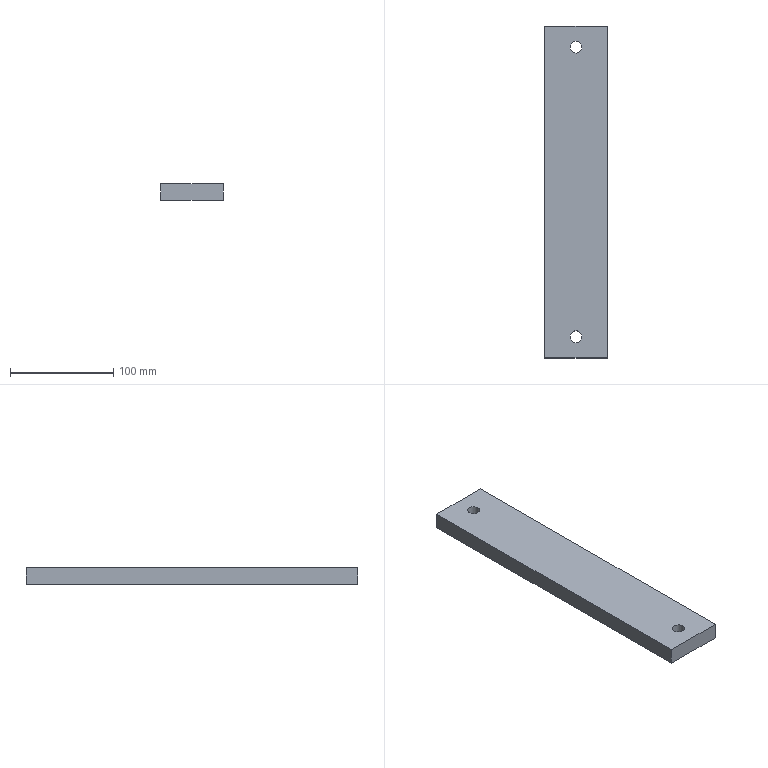Component | NX | CH3404_5-10_2 | 1 solid | 8 faces | box 60 x 321 x 16 mm | volume 304836 mm3 | plane 6 | cylinder 2 | commonest cylinder face diameters 11.5 x2
STEP:
#1=CARTESIAN_POINT('',(0.,0.,0.));
#2=DIRECTION('',(0.,0.,1.));
#3=DIRECTION('',(1.,0.,0.));
#4=AXIS2_PLACEMENT_3D('',#1,#2,#3);
#5=CARTESIAN_POINT('',(295.,-160.5,-205.));
#6=VERTEX_POINT('',#5);
#7=CARTESIAN_POINT('',(355.,-160.5,-205.));
#8=VERTEX_POINT('',#7);
#9=CARTESIAN_POINT('',(295.,-160.5,-205.));
#10=DIRECTION('',(1.,0.,0.));
#11=VECTOR('',#10,1.);
#12=LINE('',#9,#11);
#13=CARTESIAN_POINT('',(295.,-160.5,-189.));
#14=DIRECTION('',(0.,1.,0.));
#15=DIRECTION('',(0.,0.,-1.));
#16=AXIS2_PLACEMENT_3D('',#13,#14,#15);
#17=PLANE('',#16);
#18=CARTESIAN_POINT('',(16.,0.));
#19=DIRECTION('',(0.,-1.));
#20=VECTOR('',#19,1.);
#21=LINE('',#18,#20);
#22=(GEOMETRIC_REPRESENTATION_CONTEXT(2)PARAMETRIC_REPRESENTATION_CONTEXT()REPRESENTATION_CONTEXT('',''));
#23=DEFINITIONAL_REPRESENTATION('',(#21),#22);
#24=PCURVE('',#17,#23);
#25=CARTESIAN_POINT('',(325.,0.,-205.));
#26=DIRECTION('',(0.,0.,1.));
#27=DIRECTION('',(0.,1.,0.));
#28=AXIS2_PLACEMENT_3D('',#25,#26,#27);
#29=PLANE('',#28);
#30=CARTESIAN_POINT('',(-160.5,30.));
#31=DIRECTION('',(0.,-1.));
#32=VECTOR('',#31,1.);
#33=LINE('',#30,#32);
#34=(GEOMETRIC_REPRESENTATION_CONTEXT(2)PARAMETRIC_REPRESENTATION_CONTEXT()REPRESENTATION_CONTEXT('',''));
#35=DEFINITIONAL_REPRESENTATION('',(#33),#34);
#36=PCURVE('',#29,#35);
#37=SURFACE_CURVE('',#12,(#24,#36),.PCURVE_S1.);
#38=EDGE_CURVE('',#6,#8,#37,.T.);
#39=ORIENTED_EDGE('',*,*,#38,.T.);
#40=CARTESIAN_POINT('',(355.,-160.5,-189.));
#41=VERTEX_POINT('',#40);
#42=CARTESIAN_POINT('',(355.,-160.5,-189.));
#43=DIRECTION('',(0.,0.,-1.));
#44=VECTOR('',#43,1.);
#45=LINE('',#42,#44);
#46=CARTESIAN_POINT('',(0.,-60.));
#47=DIRECTION('',(1.,0.));
#48=VECTOR('',#47,1.);
#49=LINE('',#46,#48);
#50=(GEOMETRIC_REPRESENTATION_CONTEXT(2)PARAMETRIC_REPRESENTATION_CONTEXT()REPRESENTATION_CONTEXT('',''));
#51=DEFINITIONAL_REPRESENTATION('',(#49),#50);
#52=PCURVE('',#17,#51);
#53=CARTESIAN_POINT('',(355.,-160.5,-189.));
#54=DIRECTION('',(-1.,0.,0.));
#55=DIRECTION('',(0.,0.,1.));
#56=AXIS2_PLACEMENT_3D('',#53,#54,#55);
#57=PLANE('',#56);
#58=CARTESIAN_POINT('',(0.,0.));
#59=DIRECTION('',(-1.,0.));
#60=VECTOR('',#59,1.);
#61=LINE('',#58,#60);
#62=(GEOMETRIC_REPRESENTATION_CONTEXT(2)PARAMETRIC_REPRESENTATION_CONTEXT()REPRESENTATION_CONTEXT('',''));
#63=DEFINITIONAL_REPRESENTATION('',(#61),#62);
#64=PCURVE('',#57,#63);
#65=SURFACE_CURVE('',#45,(#52,#64),.PCURVE_S1.);
#66=EDGE_CURVE('',#41,#8,#65,.T.);
#67=ORIENTED_EDGE('',*,*,#66,.F.);
#68=CARTESIAN_POINT('',(295.,-160.5,-189.));
#69=VERTEX_POINT('',#68);
#70=CARTESIAN_POINT('',(295.,-160.5,-189.));
#71=DIRECTION('',(1.,0.,0.));
#72=VECTOR('',#71,1.);
#73=LINE('',#70,#72);
#74=CARTESIAN_POINT('',(0.,0.));
#75=DIRECTION('',(0.,-1.));
#76=VECTOR('',#75,1.);
#77=LINE('',#74,#76);
#78=(GEOMETRIC_REPRESENTATION_CONTEXT(2)PARAMETRIC_REPRESENTATION_CONTEXT()REPRESENTATION_CONTEXT('',''));
#79=DEFINITIONAL_REPRESENTATION('',(#77),#78);
#80=PCURVE('',#17,#79);
#81=CARTESIAN_POINT('',(325.,0.,-189.));
#82=DIRECTION('',(0.,0.,1.));
#83=DIRECTION('',(0.,1.,0.));
#84=AXIS2_PLACEMENT_3D('',#81,#82,#83);
#85=PLANE('',#84);
#86=CARTESIAN_POINT('',(-160.5,30.));
#87=DIRECTION('',(0.,-1.));
#88=VECTOR('',#87,1.);
#89=LINE('',#86,#88);
#90=(GEOMETRIC_REPRESENTATION_CONTEXT(2)PARAMETRIC_REPRESENTATION_CONTEXT()REPRESENTATION_CONTEXT('',''));
#91=DEFINITIONAL_REPRESENTATION('',(#89),#90);
#92=PCURVE('',#85,#91);
#93=SURFACE_CURVE('',#73,(#80,#92),.PCURVE_S1.);
#94=EDGE_CURVE('',#69,#41,#93,.T.);
#95=ORIENTED_EDGE('',*,*,#94,.F.);
#96=CARTESIAN_POINT('',(295.,-160.5,-189.));
#97=DIRECTION('',(0.,0.,-1.));
#98=VECTOR('',#97,1.);
#99=LINE('',#96,#98);
#100=CARTESIAN_POINT('',(0.,0.));
#101=DIRECTION('',(1.,0.));
#102=VECTOR('',#101,1.);
#103=LINE('',#100,#102);
#104=(GEOMETRIC_REPRESENTATION_CONTEXT(2)PARAMETRIC_REPRESENTATION_CONTEXT()REPRESENTATION_CONTEXT('',''));
#105=DEFINITIONAL_REPRESENTATION('',(#103),#104);
#106=PCURVE('',#17,#105);
#107=CARTESIAN_POINT('',(295.,160.5,-189.));
#108=DIRECTION('',(1.,0.,0.));
#109=DIRECTION('',(0.,0.,-1.));
#110=AXIS2_PLACEMENT_3D('',#107,#108,#109);
#111=PLANE('',#110);
#112=CARTESIAN_POINT('',(0.,-321.));
#113=DIRECTION('',(1.,0.));
#114=VECTOR('',#113,1.);
#115=LINE('',#112,#114);
#116=(GEOMETRIC_REPRESENTATION_CONTEXT(2)PARAMETRIC_REPRESENTATION_CONTEXT()REPRESENTATION_CONTEXT('',''));
#117=DEFINITIONAL_REPRESENTATION('',(#115),#116);
#118=PCURVE('',#111,#117);
#119=SURFACE_CURVE('',#99,(#106,#118),.PCURVE_S1.);
#120=EDGE_CURVE('',#69,#6,#119,.T.);
#121=ORIENTED_EDGE('',*,*,#120,.T.);
#122=EDGE_LOOP('',(#39,#67,#95,#121));
#123=FACE_BOUND('',#122,.T.);
#124=ADVANCED_FACE('',(#123),#17,.F.);
#125=CARTESIAN_POINT('',(355.,160.5,-205.));
#126=VERTEX_POINT('',#125);
#127=CARTESIAN_POINT('',(355.,-160.5,-205.));
#128=DIRECTION('',(0.,1.,0.));
#129=VECTOR('',#128,1.);
#130=LINE('',#127,#129);
#131=CARTESIAN_POINT('',(-16.,0.));
#132=DIRECTION('',(0.,1.));
#133=VECTOR('',#132,1.);
#134=LINE('',#131,#133);
#135=(GEOMETRIC_REPRESENTATION_CONTEXT(2)PARAMETRIC_REPRESENTATION_CONTEXT()REPRESENTATION_CONTEXT('',''));
#136=DEFINITIONAL_REPRESENTATION('',(#134),#135);
#137=PCURVE('',#57,#136);
#138=CARTESIAN_POINT('',(-160.5,-30.));
#139=DIRECTION('',(1.,0.));
#140=VECTOR('',#139,1.);
#141=LINE('',#138,#140);
#142=(GEOMETRIC_REPRESENTATION_CONTEXT(2)PARAMETRIC_REPRESENTATION_CONTEXT()REPRESENTATION_CONTEXT('',''));
#143=DEFINITIONAL_REPRESENTATION('',(#141),#142);
#144=PCURVE('',#29,#143);
#145=SURFACE_CURVE('',#130,(#137,#144),.PCURVE_S1.);
#146=EDGE_CURVE('',#8,#126,#145,.T.);
#147=ORIENTED_EDGE('',*,*,#146,.T.);
#148=CARTESIAN_POINT('',(355.,160.5,-189.));
#149=VERTEX_POINT('',#148);
#150=CARTESIAN_POINT('',(355.,160.5,-189.));
#151=DIRECTION('',(0.,0.,-1.));
#152=VECTOR('',#151,1.);
#153=LINE('',#150,#152);
#154=CARTESIAN_POINT('',(0.,321.));
#155=DIRECTION('',(-1.,0.));
#156=VECTOR('',#155,1.);
#157=LINE('',#154,#156);
#158=(GEOMETRIC_REPRESENTATION_CONTEXT(2)PARAMETRIC_REPRESENTATION_CONTEXT()REPRESENTATION_CONTEXT('',''));
#159=DEFINITIONAL_REPRESENTATION('',(#157),#158);
#160=PCURVE('',#57,#159);
#161=CARTESIAN_POINT('',(355.,160.5,-189.));
#162=DIRECTION('',(0.,-1.,0.));
#163=DIRECTION('',(0.,0.,1.));
#164=AXIS2_PLACEMENT_3D('',#161,#162,#163);
#165=PLANE('',#164);
#166=CARTESIAN_POINT('',(0.,0.));
#167=DIRECTION('',(-1.,0.));
#168=VECTOR('',#167,1.);
#169=LINE('',#166,#168);
#170=(GEOMETRIC_REPRESENTATION_CONTEXT(2)PARAMETRIC_REPRESENTATION_CONTEXT()REPRESENTATION_CONTEXT('',''));
#171=DEFINITIONAL_REPRESENTATION('',(#169),#170);
#172=PCURVE('',#165,#171);
#173=SURFACE_CURVE('',#153,(#160,#172),.PCURVE_S1.);
#174=EDGE_CURVE('',#149,#126,#173,.T.);
#175=ORIENTED_EDGE('',*,*,#174,.F.);
#176=CARTESIAN_POINT('',(355.,-160.5,-189.));
#177=DIRECTION('',(0.,1.,0.));
#178=VECTOR('',#177,1.);
#179=LINE('',#176,#178);
#180=CARTESIAN_POINT('',(0.,0.));
#181=DIRECTION('',(0.,1.));
#182=VECTOR('',#181,1.);
#183=LINE('',#180,#182);
#184=(GEOMETRIC_REPRESENTATION_CONTEXT(2)PARAMETRIC_REPRESENTATION_CONTEXT()REPRESENTATION_CONTEXT('',''));
#185=DEFINITIONAL_REPRESENTATION('',(#183),#184);
#186=PCURVE('',#57,#185);
#187=CARTESIAN_POINT('',(-160.5,-30.));
#188=DIRECTION('',(1.,0.));
#189=VECTOR('',#188,1.);
#190=LINE('',#187,#189);
#191=(GEOMETRIC_REPRESENTATION_CONTEXT(2)PARAMETRIC_REPRESENTATION_CONTEXT()REPRESENTATION_CONTEXT('',''));
#192=DEFINITIONAL_REPRESENTATION('',(#190),#191);
#193=PCURVE('',#85,#192);
#194=SURFACE_CURVE('',#179,(#186,#193),.PCURVE_S1.);
#195=EDGE_CURVE('',#41,#149,#194,.T.);
#196=ORIENTED_EDGE('',*,*,#195,.F.);
#197=ORIENTED_EDGE('',*,*,#66,.T.);
#198=EDGE_LOOP('',(#147,#175,#196,#197));
#199=FACE_BOUND('',#198,.T.);
#200=ADVANCED_FACE('',(#199),#57,.F.);
#201=CARTESIAN_POINT('',(295.,160.5,-205.));
#202=VERTEX_POINT('',#201);
#203=CARTESIAN_POINT('',(355.,160.5,-205.));
#204=DIRECTION('',(-1.,0.,0.));
#205=VECTOR('',#204,1.);
#206=LINE('',#203,#205);
#207=CARTESIAN_POINT('',(-16.,0.));
#208=DIRECTION('',(0.,1.));
#209=VECTOR('',#208,1.);
#210=LINE('',#207,#209);
#211=(GEOMETRIC_REPRESENTATION_CONTEXT(2)PARAMETRIC_REPRESENTATION_CONTEXT()REPRESENTATION_CONTEXT('',''));
#212=DEFINITIONAL_REPRESENTATION('',(#210),#211);
#213=PCURVE('',#165,#212);
#214=CARTESIAN_POINT('',(160.5,-30.));
#215=DIRECTION('',(0.,1.));
#216=VECTOR('',#215,1.);
#217=LINE('',#214,#216);
#218=(GEOMETRIC_REPRESENTATION_CONTEXT(2)PARAMETRIC_REPRESENTATION_CONTEXT()REPRESENTATION_CONTEXT('',''));
#219=DEFINITIONAL_REPRESENTATION('',(#217),#218);
#220=PCURVE('',#29,#219);
#221=SURFACE_CURVE('',#206,(#213,#220),.PCURVE_S1.);
#222=EDGE_CURVE('',#126,#202,#221,.T.);
#223=ORIENTED_EDGE('',*,*,#222,.T.);
#224=CARTESIAN_POINT('',(295.,160.5,-189.));
#225=VERTEX_POINT('',#224);
#226=CARTESIAN_POINT('',(295.,160.5,-189.));
#227=DIRECTION('',(0.,0.,-1.));
#228=VECTOR('',#227,1.);
#229=LINE('',#226,#228);
#230=CARTESIAN_POINT('',(0.,60.));
#231=DIRECTION('',(-1.,0.));
#232=VECTOR('',#231,1.);
#233=LINE('',#230,#232);
#234=(GEOMETRIC_REPRESENTATION_CONTEXT(2)PARAMETRIC_REPRESENTATION_CONTEXT()REPRESENTATION_CONTEXT('',''));
#235=DEFINITIONAL_REPRESENTATION('',(#233),#234);
#236=PCURVE('',#165,#235);
#237=CARTESIAN_POINT('',(0.,0.));
#238=DIRECTION('',(1.,0.));
#239=VECTOR('',#238,1.);
#240=LINE('',#237,#239);
#241=(GEOMETRIC_REPRESENTATION_CONTEXT(2)PARAMETRIC_REPRESENTATION_CONTEXT()REPRESENTATION_CONTEXT('',''));
#242=DEFINITIONAL_REPRESENTATION('',(#240),#241);
#243=PCURVE('',#111,#242);
#244=SURFACE_CURVE('',#229,(#236,#243),.PCURVE_S1.);
#245=EDGE_CURVE('',#225,#202,#244,.T.);
#246=ORIENTED_EDGE('',*,*,#245,.F.);
#247=CARTESIAN_POINT('',(355.,160.5,-189.));
#248=DIRECTION('',(-1.,0.,0.));
#249=VECTOR('',#248,1.);
#250=LINE('',#247,#249);
#251=CARTESIAN_POINT('',(0.,0.));
#252=DIRECTION('',(0.,1.));
#253=VECTOR('',#252,1.);
#254=LINE('',#251,#253);
#255=(GEOMETRIC_REPRESENTATION_CONTEXT(2)PARAMETRIC_REPRESENTATION_CONTEXT()REPRESENTATION_CONTEXT('',''));
#256=DEFINITIONAL_REPRESENTATION('',(#254),#255);
#257=PCURVE('',#165,#256);
#258=CARTESIAN_POINT('',(160.5,-30.));
#259=DIRECTION('',(0.,1.));
#260=VECTOR('',#259,1.);
#261=LINE('',#258,#260);
#262=(GEOMETRIC_REPRESENTATION_CONTEXT(2)PARAMETRIC_REPRESENTATION_CONTEXT()REPRESENTATION_CONTEXT('',''));
#263=DEFINITIONAL_REPRESENTATION('',(#261),#262);
#264=PCURVE('',#85,#263);
#265=SURFACE_CURVE('',#250,(#257,#264),.PCURVE_S1.);
#266=EDGE_CURVE('',#149,#225,#265,.T.);
#267=ORIENTED_EDGE('',*,*,#266,.F.);
#268=ORIENTED_EDGE('',*,*,#174,.T.);
#269=EDGE_LOOP('',(#223,#246,#267,#268));
#270=FACE_BOUND('',#269,.T.);
#271=ADVANCED_FACE('',(#270),#165,.F.);
#272=CARTESIAN_POINT('',(295.,160.5,-205.));
#273=DIRECTION('',(0.,-1.,0.));
#274=VECTOR('',#273,1.);
#275=LINE('',#272,#274);
#276=CARTESIAN_POINT('',(16.,0.));
#277=DIRECTION('',(0.,-1.));
#278=VECTOR('',#277,1.);
#279=LINE('',#276,#278);
#280=(GEOMETRIC_REPRESENTATION_CONTEXT(2)PARAMETRIC_REPRESENTATION_CONTEXT()REPRESENTATION_CONTEXT('',''));
#281=DEFINITIONAL_REPRESENTATION('',(#279),#280);
#282=PCURVE('',#111,#281);
#283=CARTESIAN_POINT('',(160.5,30.));
#284=DIRECTION('',(-1.,0.));
#285=VECTOR('',#284,1.);
#286=LINE('',#283,#285);
#287=(GEOMETRIC_REPRESENTATION_CONTEXT(2)PARAMETRIC_REPRESENTATION_CONTEXT()REPRESENTATION_CONTEXT('',''));
#288=DEFINITIONAL_REPRESENTATION('',(#286),#287);
#289=PCURVE('',#29,#288);
#290=SURFACE_CURVE('',#275,(#282,#289),.PCURVE_S1.);
#291=EDGE_CURVE('',#202,#6,#290,.T.);
#292=ORIENTED_EDGE('',*,*,#291,.T.);
#293=ORIENTED_EDGE('',*,*,#120,.F.);
#294=CARTESIAN_POINT('',(295.,160.5,-189.));
#295=DIRECTION('',(0.,-1.,0.));
#296=VECTOR('',#295,1.);
#297=LINE('',#294,#296);
#298=CARTESIAN_POINT('',(0.,0.));
#299=DIRECTION('',(0.,-1.));
#300=VECTOR('',#299,1.);
#301=LINE('',#298,#300);
#302=(GEOMETRIC_REPRESENTATION_CONTEXT(2)PARAMETRIC_REPRESENTATION_CONTEXT()REPRESENTATION_CONTEXT('',''));
#303=DEFINITIONAL_REPRESENTATION('',(#301),#302);
#304=PCURVE('',#111,#303);
#305=CARTESIAN_POINT('',(160.5,30.));
#306=DIRECTION('',(-1.,0.));
#307=VECTOR('',#306,1.);
#308=LINE('',#305,#307);
#309=(GEOMETRIC_REPRESENTATION_CONTEXT(2)PARAMETRIC_REPRESENTATION_CONTEXT()REPRESENTATION_CONTEXT('',''));
#310=DEFINITIONAL_REPRESENTATION('',(#308),#309);
#311=PCURVE('',#85,#310);
#312=SURFACE_CURVE('',#297,(#304,#311),.PCURVE_S1.);
#313=EDGE_CURVE('',#225,#69,#312,.T.);
#314=ORIENTED_EDGE('',*,*,#313,.F.);
#315=ORIENTED_EDGE('',*,*,#245,.T.);
#316=EDGE_LOOP('',(#292,#293,#314,#315));
#317=FACE_BOUND('',#316,.T.);
#318=ADVANCED_FACE('',(#317),#111,.F.);
#319=CARTESIAN_POINT('',(325.,134.25,-189.));
#320=VERTEX_POINT('',#319);
#321=CARTESIAN_POINT('',(325.,140.,-189.));
#322=DIRECTION('',(0.,0.,-1.));
#323=DIRECTION('',(0.,-1.,0.));
#324=AXIS2_PLACEMENT_3D('',#321,#322,#323);
#325=CIRCLE('',#324,5.75);
#326=CARTESIAN_POINT('',(134.25,0.));
#327=CARTESIAN_POINT('',(134.25,9.959));
#328=CARTESIAN_POINT('',(142.875,4.98));
#329=CARTESIAN_POINT('',(151.5,0.));
#330=CARTESIAN_POINT('',(142.875,-4.98));
#331=CARTESIAN_POINT('',(134.25,-9.959));
#332=CARTESIAN_POINT('',(134.25,0.));
#333=(BOUNDED_CURVE()B_SPLINE_CURVE(2,(#326,#327,#328,#329,#330,#331,#332),.UNSPECIFIED.,.T.,.F.)B_SPLINE_CURVE_WITH_KNOTS((1,2,2,2,2,1),(-2.094,0.,2.094,4.189,6.283,8.378),.UNSPECIFIED.)CURVE()GEOMETRIC_REPRESENTATION_ITEM()RATIONAL_B_SPLINE_CURVE((1.,0.5,1.,0.5,1.,0.5,1.))REPRESENTATION_ITEM(''));
#334=(GEOMETRIC_REPRESENTATION_CONTEXT(2)PARAMETRIC_REPRESENTATION_CONTEXT()REPRESENTATION_CONTEXT('',''));
#335=DEFINITIONAL_REPRESENTATION('',(#333),#334);
#336=PCURVE('',#85,#335);
#337=CARTESIAN_POINT('',(325.,140.,-189.));
#338=DIRECTION('',(0.,0.,-1.));
#339=DIRECTION('',(0.,-1.,0.));
#340=AXIS2_PLACEMENT_3D('',#337,#338,#339);
#341=CYLINDRICAL_SURFACE('',#340,5.75);
#342=CARTESIAN_POINT('',(0.,0.));
#343=DIRECTION('',(1.,0.));
#344=VECTOR('',#343,1.);
#345=LINE('',#342,#344);
#346=(GEOMETRIC_REPRESENTATION_CONTEXT(2)PARAMETRIC_REPRESENTATION_CONTEXT()REPRESENTATION_CONTEXT('',''));
#347=DEFINITIONAL_REPRESENTATION('',(#345),#346);
#348=PCURVE('',#341,#347);
#349=SURFACE_CURVE('',#325,(#336,#348),.PCURVE_S1.);
#350=EDGE_CURVE('',#320,#320,#349,.T.);
#351=ORIENTED_EDGE('',*,*,#350,.T.);
#352=EDGE_LOOP('',(#351));
#353=FACE_BOUND('',#352,.T.);
#354=CARTESIAN_POINT('',(325.,-145.75,-189.));
#355=VERTEX_POINT('',#354);
#356=CARTESIAN_POINT('',(325.,-140.,-189.));
#357=DIRECTION('',(0.,0.,-1.));
#358=DIRECTION('',(0.,-1.,0.));
#359=AXIS2_PLACEMENT_3D('',#356,#357,#358);
#360=CIRCLE('',#359,5.75);
#361=CARTESIAN_POINT('',(-145.75,0.));
#362=CARTESIAN_POINT('',(-145.75,9.959));
#363=CARTESIAN_POINT('',(-137.125,4.98));
#364=CARTESIAN_POINT('',(-128.5,0.));
#365=CARTESIAN_POINT('',(-137.125,-4.98));
#366=CARTESIAN_POINT('',(-145.75,-9.959));
#367=CARTESIAN_POINT('',(-145.75,0.));
#368=(BOUNDED_CURVE()B_SPLINE_CURVE(2,(#361,#362,#363,#364,#365,#366,#367),.UNSPECIFIED.,.T.,.F.)B_SPLINE_CURVE_WITH_KNOTS((1,2,2,2,2,1),(-2.094,0.,2.094,4.189,6.283,8.378),.UNSPECIFIED.)CURVE()GEOMETRIC_REPRESENTATION_ITEM()RATIONAL_B_SPLINE_CURVE((1.,0.5,1.,0.5,1.,0.5,1.))REPRESENTATION_ITEM(''));
#369=(GEOMETRIC_REPRESENTATION_CONTEXT(2)PARAMETRIC_REPRESENTATION_CONTEXT()REPRESENTATION_CONTEXT('',''));
#370=DEFINITIONAL_REPRESENTATION('',(#368),#369);
#371=PCURVE('',#85,#370);
#372=CARTESIAN_POINT('',(325.,-140.,-189.));
#373=DIRECTION('',(0.,0.,-1.));
#374=DIRECTION('',(0.,-1.,0.));
#375=AXIS2_PLACEMENT_3D('',#372,#373,#374);
#376=CYLINDRICAL_SURFACE('',#375,5.75);
#377=CARTESIAN_POINT('',(0.,0.));
#378=DIRECTION('',(1.,0.));
#379=VECTOR('',#378,1.);
#380=LINE('',#377,#379);
#381=(GEOMETRIC_REPRESENTATION_CONTEXT(2)PARAMETRIC_REPRESENTATION_CONTEXT()REPRESENTATION_CONTEXT('',''));
#382=DEFINITIONAL_REPRESENTATION('',(#380),#381);
#383=PCURVE('',#376,#382);
#384=SURFACE_CURVE('',#360,(#371,#383),.PCURVE_S1.);
#385=EDGE_CURVE('',#355,#355,#384,.T.);
#386=ORIENTED_EDGE('',*,*,#385,.T.);
#387=EDGE_LOOP('',(#386));
#388=FACE_BOUND('',#387,.T.);
#389=ORIENTED_EDGE('',*,*,#94,.T.);
#390=ORIENTED_EDGE('',*,*,#195,.T.);
#391=ORIENTED_EDGE('',*,*,#266,.T.);
#392=ORIENTED_EDGE('',*,*,#313,.T.);
#393=EDGE_LOOP('',(#389,#390,#391,#392));
#394=FACE_BOUND('',#393,.T.);
#395=ADVANCED_FACE('',(#353,#388,#394),#85,.T.);
#396=CARTESIAN_POINT('',(325.,145.75,-205.));
#397=VERTEX_POINT('',#396);
#398=CARTESIAN_POINT('',(325.,134.25,-205.));
#399=VERTEX_POINT('',#398);
#400=CARTESIAN_POINT('',(325.,140.,-205.));
#401=DIRECTION('',(0.,0.,1.));
#402=DIRECTION('',(0.,1.,0.));
#403=AXIS2_PLACEMENT_3D('',#400,#401,#402);
#404=CIRCLE('',#403,5.75);
#405=CARTESIAN_POINT('',(140.,0.));
#406=DIRECTION('',(1.,0.));
#407=AXIS2_PLACEMENT_2D('',#405,#406);
#408=CIRCLE('',#407,5.75);
#409=(GEOMETRIC_REPRESENTATION_CONTEXT(2)PARAMETRIC_REPRESENTATION_CONTEXT()REPRESENTATION_CONTEXT('',''));
#410=DEFINITIONAL_REPRESENTATION('',(#408),#409);
#411=PCURVE('',#29,#410);
#412=CARTESIAN_POINT('',(3.142,16.));
#413=DIRECTION('',(-1.,0.));
#414=VECTOR('',#413,1.);
#415=LINE('',#412,#414);
#416=(GEOMETRIC_REPRESENTATION_CONTEXT(2)PARAMETRIC_REPRESENTATION_CONTEXT()REPRESENTATION_CONTEXT('',''));
#417=DEFINITIONAL_REPRESENTATION('',(#415),#416);
#418=PCURVE('',#341,#417);
#419=SURFACE_CURVE('',#404,(#411,#418),.PCURVE_S1.);
#420=EDGE_CURVE('',#397,#399,#419,.T.);
#421=ORIENTED_EDGE('',*,*,#420,.T.);
#422=CARTESIAN_POINT('',(325.,140.,-205.));
#423=DIRECTION('',(0.,0.,1.));
#424=DIRECTION('',(0.,1.,0.));
#425=AXIS2_PLACEMENT_3D('',#422,#423,#424);
#426=CIRCLE('',#425,5.75);
#427=CARTESIAN_POINT('',(140.,0.));
#428=DIRECTION('',(1.,0.));
#429=AXIS2_PLACEMENT_2D('',#427,#428);
#430=CIRCLE('',#429,5.75);
#431=(GEOMETRIC_REPRESENTATION_CONTEXT(2)PARAMETRIC_REPRESENTATION_CONTEXT()REPRESENTATION_CONTEXT('',''));
#432=DEFINITIONAL_REPRESENTATION('',(#430),#431);
#433=PCURVE('',#29,#432);
#434=CARTESIAN_POINT('',(9.425,16.));
#435=DIRECTION('',(-1.,0.));
#436=VECTOR('',#435,1.);
#437=LINE('',#434,#436);
#438=(GEOMETRIC_REPRESENTATION_CONTEXT(2)PARAMETRIC_REPRESENTATION_CONTEXT()REPRESENTATION_CONTEXT('',''));
#439=DEFINITIONAL_REPRESENTATION('',(#437),#438);
#440=PCURVE('',#341,#439);
#441=SURFACE_CURVE('',#426,(#433,#440),.PCURVE_S1.);
#442=EDGE_CURVE('',#399,#397,#441,.T.);
#443=ORIENTED_EDGE('',*,*,#442,.T.);
#444=EDGE_LOOP('',(#421,#443));
#445=FACE_BOUND('',#444,.T.);
#446=CARTESIAN_POINT('',(325.,-134.25,-205.));
#447=VERTEX_POINT('',#446);
#448=CARTESIAN_POINT('',(325.,-145.75,-205.));
#449=VERTEX_POINT('',#448);
#450=CARTESIAN_POINT('',(325.,-140.,-205.));
#451=DIRECTION('',(0.,0.,1.));
#452=DIRECTION('',(0.,1.,0.));
#453=AXIS2_PLACEMENT_3D('',#450,#451,#452);
#454=CIRCLE('',#453,5.75);
#455=CARTESIAN_POINT('',(-140.,0.));
#456=DIRECTION('',(1.,0.));
#457=AXIS2_PLACEMENT_2D('',#455,#456);
#458=CIRCLE('',#457,5.75);
#459=(GEOMETRIC_REPRESENTATION_CONTEXT(2)PARAMETRIC_REPRESENTATION_CONTEXT()REPRESENTATION_CONTEXT('',''));
#460=DEFINITIONAL_REPRESENTATION('',(#458),#459);
#461=PCURVE('',#29,#460);
#462=CARTESIAN_POINT('',(3.142,16.));
#463=DIRECTION('',(-1.,0.));
#464=VECTOR('',#463,1.);
#465=LINE('',#462,#464);
#466=(GEOMETRIC_REPRESENTATION_CONTEXT(2)PARAMETRIC_REPRESENTATION_CONTEXT()REPRESENTATION_CONTEXT('',''));
#467=DEFINITIONAL_REPRESENTATION('',(#465),#466);
#468=PCURVE('',#376,#467);
#469=SURFACE_CURVE('',#454,(#461,#468),.PCURVE_S1.);
#470=EDGE_CURVE('',#447,#449,#469,.T.);
#471=ORIENTED_EDGE('',*,*,#470,.T.);
#472=CARTESIAN_POINT('',(325.,-140.,-205.));
#473=DIRECTION('',(0.,0.,1.));
#474=DIRECTION('',(0.,1.,0.));
#475=AXIS2_PLACEMENT_3D('',#472,#473,#474);
#476=CIRCLE('',#475,5.75);
#477=CARTESIAN_POINT('',(-140.,0.));
#478=DIRECTION('',(1.,0.));
#479=AXIS2_PLACEMENT_2D('',#477,#478);
#480=CIRCLE('',#479,5.75);
#481=(GEOMETRIC_REPRESENTATION_CONTEXT(2)PARAMETRIC_REPRESENTATION_CONTEXT()REPRESENTATION_CONTEXT('',''));
#482=DEFINITIONAL_REPRESENTATION('',(#480),#481);
#483=PCURVE('',#29,#482);
#484=CARTESIAN_POINT('',(9.425,16.));
#485=DIRECTION('',(-1.,0.));
#486=VECTOR('',#485,1.);
#487=LINE('',#484,#486);
#488=(GEOMETRIC_REPRESENTATION_CONTEXT(2)PARAMETRIC_REPRESENTATION_CONTEXT()REPRESENTATION_CONTEXT('',''));
#489=DEFINITIONAL_REPRESENTATION('',(#487),#488);
#490=PCURVE('',#376,#489);
#491=SURFACE_CURVE('',#476,(#483,#490),.PCURVE_S1.);
#492=EDGE_CURVE('',#449,#447,#491,.T.);
#493=ORIENTED_EDGE('',*,*,#492,.T.);
#494=EDGE_LOOP('',(#471,#493));
#495=FACE_BOUND('',#494,.T.);
#496=ORIENTED_EDGE('',*,*,#38,.F.);
#497=ORIENTED_EDGE('',*,*,#291,.F.);
#498=ORIENTED_EDGE('',*,*,#222,.F.);
#499=ORIENTED_EDGE('',*,*,#146,.F.);
#500=EDGE_LOOP('',(#496,#497,#498,#499));
#501=FACE_BOUND('',#500,.T.);
#502=ADVANCED_FACE('',(#445,#495,#501),#29,.F.);
#503=ORIENTED_EDGE('',*,*,#385,.T.);
#504=CARTESIAN_POINT('',(325.,-145.75,-189.));
#505=CARTESIAN_POINT('',(325.,-145.75,-205.));
#506=B_SPLINE_CURVE_WITH_KNOTS('',1,(#504,#505),.UNSPECIFIED.,.F.,.F.,(2,2),(0.,16.),.PIECEWISE_BEZIER_KNOTS.);
#507=CARTESIAN_POINT('',(6.283,0.));
#508=DIRECTION('',(0.,1.));
#509=VECTOR('',#508,1.);
#510=LINE('',#507,#509);
#511=(GEOMETRIC_REPRESENTATION_CONTEXT(2)PARAMETRIC_REPRESENTATION_CONTEXT()REPRESENTATION_CONTEXT('',''));
#512=DEFINITIONAL_REPRESENTATION('',(#510),#511);
#513=PCURVE('',#376,#512);
#514=CARTESIAN_POINT('',(0.,0.));
#515=DIRECTION('',(0.,1.));
#516=VECTOR('',#515,1.);
#517=LINE('',#514,#516);
#518=(GEOMETRIC_REPRESENTATION_CONTEXT(2)PARAMETRIC_REPRESENTATION_CONTEXT()REPRESENTATION_CONTEXT('',''));
#519=DEFINITIONAL_REPRESENTATION('',(#517),#518);
#520=PCURVE('',#376,#519);
#521=SEAM_CURVE('',#506,(#513,#520),.PCURVE_S1.);
#522=EDGE_CURVE('',#355,#449,#521,.T.);
#523=ORIENTED_EDGE('',*,*,#522,.T.);
#524=ORIENTED_EDGE('',*,*,#492,.T.);
#525=ORIENTED_EDGE('',*,*,#470,.T.);
#526=ORIENTED_EDGE('',*,*,#522,.F.);
#527=EDGE_LOOP('',(#503,#523,#524,#525,#526));
#528=FACE_BOUND('',#527,.F.);
#529=ADVANCED_FACE('',(#528),#376,.F.);
#530=ORIENTED_EDGE('',*,*,#350,.T.);
#531=CARTESIAN_POINT('',(325.,134.25,-189.));
#532=CARTESIAN_POINT('',(325.,134.25,-205.));
#533=B_SPLINE_CURVE_WITH_KNOTS('',1,(#531,#532),.UNSPECIFIED.,.F.,.F.,(2,2),(0.,16.),.PIECEWISE_BEZIER_KNOTS.);
#534=CARTESIAN_POINT('',(6.283,0.));
#535=DIRECTION('',(0.,1.));
#536=VECTOR('',#535,1.);
#537=LINE('',#534,#536);
#538=(GEOMETRIC_REPRESENTATION_CONTEXT(2)PARAMETRIC_REPRESENTATION_CONTEXT()REPRESENTATION_CONTEXT('',''));
#539=DEFINITIONAL_REPRESENTATION('',(#537),#538);
#540=PCURVE('',#341,#539);
#541=CARTESIAN_POINT('',(0.,0.));
#542=DIRECTION('',(0.,1.));
#543=VECTOR('',#542,1.);
#544=LINE('',#541,#543);
#545=(GEOMETRIC_REPRESENTATION_CONTEXT(2)PARAMETRIC_REPRESENTATION_CONTEXT()REPRESENTATION_CONTEXT('',''));
#546=DEFINITIONAL_REPRESENTATION('',(#544),#545);
#547=PCURVE('',#341,#546);
#548=SEAM_CURVE('',#533,(#540,#547),.PCURVE_S1.);
#549=EDGE_CURVE('',#320,#399,#548,.T.);
#550=ORIENTED_EDGE('',*,*,#549,.T.);
#551=ORIENTED_EDGE('',*,*,#442,.T.);
#552=ORIENTED_EDGE('',*,*,#420,.T.);
#553=ORIENTED_EDGE('',*,*,#549,.F.);
#554=EDGE_LOOP('',(#530,#550,#551,#552,#553));
#555=FACE_BOUND('',#554,.F.);
#556=ADVANCED_FACE('',(#555),#341,.F.);
#557=CLOSED_SHELL('',(#124,#200,#271,#318,#395,#502,#529,#556));
#558=MANIFOLD_SOLID_BREP('',#557);
#559=(LENGTH_UNIT()NAMED_UNIT(*)SI_UNIT(.MILLI.,.METRE.));
#560=UNCERTAINTY_MEASURE_WITH_UNIT(LENGTH_MEASURE(0.000002),#559,'','');
#561=(NAMED_UNIT(*)PLANE_ANGLE_UNIT()SI_UNIT($,.RADIAN.));
#562=(NAMED_UNIT(*)SI_UNIT($,.STERADIAN.)SOLID_ANGLE_UNIT());
#563=(GEOMETRIC_REPRESENTATION_CONTEXT(3)GLOBAL_UNCERTAINTY_ASSIGNED_CONTEXT((#560))GLOBAL_UNIT_ASSIGNED_CONTEXT((#559,#561,#562))REPRESENTATION_CONTEXT('',''));
#564=ADVANCED_BREP_SHAPE_REPRESENTATION('',(#4,#558),#563);